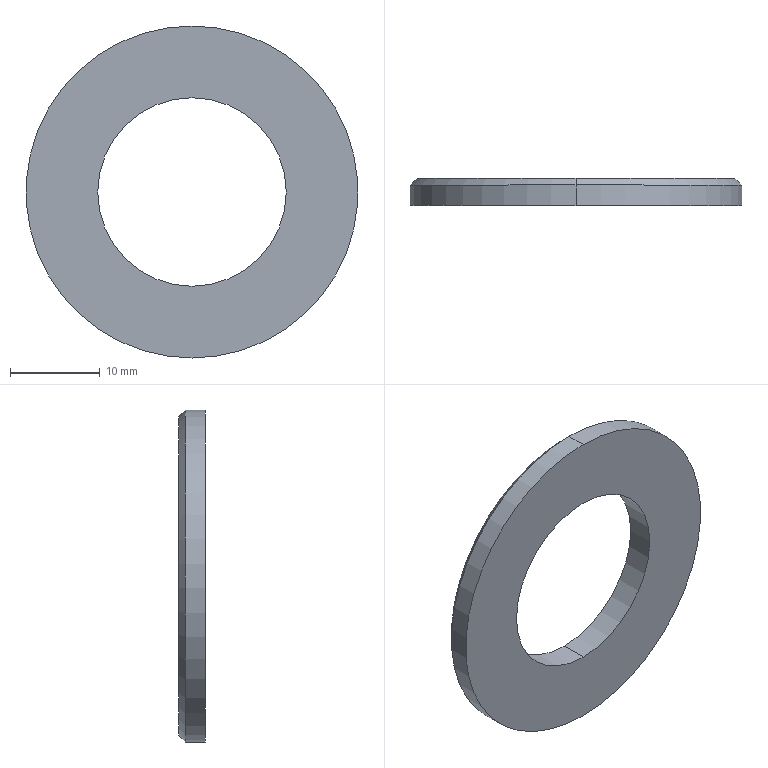Component | SolidWorks | GB_T97.2-1985FlatWasherChamferedTypeA-grade20_3-3 | 1 solid | 8 faces | box 37 x 3 x 37 mm | volume 2154 mm3 | cylinder 4 | cone 2 | plane 2 | commonest cylinder face diameters 37 x2 21 x2
build123d program:
from build123d import *


with BuildPart() as part:
    # Sketch1 → Base-Revolve (revolve)
    with BuildSketch(Plane.XY, mode=Mode.PRIVATE) as base_revolve_sk:
        Polygon((-17.75, 11.645), (-18.5, 10.895), (-18.5, 8.645), (-10.5, 8.645), (-10.5, 11.645), align=None)
    revolve(base_revolve_sk.sketch.rotate(Axis((0, 0, 0), (0, 1, 0)), 270), axis=Axis((0, 0, 0), (0, 1, 0)))


solid = part.part

# Placed as in the assembly
solid = solid.moved(Location((180, -200.645, 130), (0, 0, 0)))
STEP:
#1=CARTESIAN_POINT('',(7.087,-7.47,4.39));
#2=VERTEX_POINT('',#1);
#3=CARTESIAN_POINT('',(7.087,-7.47,5.846));
#4=VERTEX_POINT('',#3);
#5=CARTESIAN_POINT('',(7.087,-7.47,5.118));
#6=DIRECTION('',(0.,-1.,0.));
#7=DIRECTION('',(0.,0.,-1.));
#8=AXIS2_PLACEMENT_3D('',#5,#6,#7);
#9=CIRCLE('',#8,0.7283);
#10=EDGE_CURVE('',#2,#4,#9,.T.);
#11=ORIENTED_EDGE('',*,*,#10,.T.);
#12=CARTESIAN_POINT('',(7.087,-7.559,5.846));
#13=VERTEX_POINT('',#12);
#14=CARTESIAN_POINT('',(7.087,-7.899,5.846));
#15=DIRECTION('',(0.,-1.,0.));
#16=VECTOR('',#15,39.37);
#17=LINE('',#14,#16);
#18=EDGE_CURVE('',#4,#13,#17,.T.);
#19=ORIENTED_EDGE('',*,*,#18,.T.);
#20=CARTESIAN_POINT('',(7.087,-7.559,4.39));
#21=VERTEX_POINT('',#20);
#22=CARTESIAN_POINT('',(7.087,-7.559,5.118));
#23=DIRECTION('',(0.,-1.,0.));
#24=DIRECTION('',(0.,0.,-1.));
#25=AXIS2_PLACEMENT_3D('',#22,#23,#24);
#26=CIRCLE('',#25,0.7283);
#27=EDGE_CURVE('',#21,#13,#26,.T.);
#28=ORIENTED_EDGE('',*,*,#27,.F.);
#29=CARTESIAN_POINT('',(7.087,-7.899,4.39));
#30=DIRECTION('',(0.,-1.,0.));
#31=VECTOR('',#30,39.37);
#32=LINE('',#29,#31);
#33=EDGE_CURVE('',#2,#21,#32,.T.);
#34=ORIENTED_EDGE('',*,*,#33,.F.);
#35=EDGE_LOOP('',(#11,#19,#28,#34));
#36=FACE_OUTER_BOUND('',#35,.T.);
#37=CARTESIAN_POINT('',(7.087,-7.899,5.118));
#38=DIRECTION('',(0.,-1.,0.));
#39=DIRECTION('',(0.,0.,-1.));
#40=AXIS2_PLACEMENT_3D('',#37,#38,#39);
#41=CYLINDRICAL_SURFACE('',#40,0.7283);
#42=ADVANCED_FACE('',(#36),#41,.T.);
#43=CARTESIAN_POINT('',(7.087,-7.441,4.419));
#44=VERTEX_POINT('',#43);
#45=CARTESIAN_POINT('',(7.087,-7.441,5.817));
#46=VERTEX_POINT('',#45);
#47=CARTESIAN_POINT('',(7.087,-7.441,5.118));
#48=DIRECTION('',(0.,-1.,0.));
#49=DIRECTION('',(0.,0.,-1.));
#50=AXIS2_PLACEMENT_3D('',#47,#48,#49);
#51=CIRCLE('',#50,0.6988);
#52=EDGE_CURVE('',#44,#46,#51,.T.);
#53=ORIENTED_EDGE('',*,*,#52,.T.);
#54=CARTESIAN_POINT('',(7.087,-7.441,5.817));
#55=DIRECTION('',(0.,-0.7071,0.7071));
#56=VECTOR('',#55,39.37);
#57=LINE('',#54,#56);
#58=EDGE_CURVE('',#46,#4,#57,.T.);
#59=ORIENTED_EDGE('',*,*,#58,.T.);
#60=ORIENTED_EDGE('',*,*,#10,.F.);
#61=CARTESIAN_POINT('',(7.087,-7.441,4.419));
#62=DIRECTION('',(0.,-0.7071,-0.7071));
#63=VECTOR('',#62,39.37);
#64=LINE('',#61,#63);
#65=EDGE_CURVE('',#44,#2,#64,.T.);
#66=ORIENTED_EDGE('',*,*,#65,.F.);
#67=EDGE_LOOP('',(#53,#59,#60,#66));
#68=FACE_OUTER_BOUND('',#67,.T.);
#69=CARTESIAN_POINT('',(7.087,-7.441,5.118));
#70=DIRECTION('',(0.,-1.,0.));
#71=DIRECTION('',(0.,0.,-1.));
#72=AXIS2_PLACEMENT_3D('',#69,#70,#71);
#73=CONICAL_SURFACE('',#72,0.6988,0.7854);
#74=ADVANCED_FACE('',(#68),#73,.T.);
#75=CARTESIAN_POINT('',(7.087,-7.441,5.531));
#76=VERTEX_POINT('',#75);
#77=CARTESIAN_POINT('',(7.087,-7.441,4.705));
#78=VERTEX_POINT('',#77);
#79=CARTESIAN_POINT('',(7.087,-7.441,5.118));
#80=DIRECTION('',(0.,-1.,0.));
#81=DIRECTION('',(0.,0.,-1.));
#82=AXIS2_PLACEMENT_3D('',#79,#80,#81);
#83=CIRCLE('',#82,0.4134);
#84=EDGE_CURVE('',#76,#78,#83,.T.);
#85=ORIENTED_EDGE('',*,*,#84,.F.);
#86=CARTESIAN_POINT('',(7.087,-7.559,5.531));
#87=VERTEX_POINT('',#86);
#88=CARTESIAN_POINT('',(7.087,-7.899,5.531));
#89=DIRECTION('',(0.,-1.,0.));
#90=VECTOR('',#89,39.37);
#91=LINE('',#88,#90);
#92=EDGE_CURVE('',#76,#87,#91,.T.);
#93=ORIENTED_EDGE('',*,*,#92,.T.);
#94=CARTESIAN_POINT('',(7.087,-7.559,4.705));
#95=VERTEX_POINT('',#94);
#96=CARTESIAN_POINT('',(7.087,-7.559,5.118));
#97=DIRECTION('',(0.,-1.,0.));
#98=DIRECTION('',(0.,0.,-1.));
#99=AXIS2_PLACEMENT_3D('',#96,#97,#98);
#100=CIRCLE('',#99,0.4134);
#101=EDGE_CURVE('',#87,#95,#100,.T.);
#102=ORIENTED_EDGE('',*,*,#101,.T.);
#103=CARTESIAN_POINT('',(7.087,-7.899,4.705));
#104=DIRECTION('',(0.,-1.,0.));
#105=VECTOR('',#104,39.37);
#106=LINE('',#103,#105);
#107=EDGE_CURVE('',#78,#95,#106,.T.);
#108=ORIENTED_EDGE('',*,*,#107,.F.);
#109=EDGE_LOOP('',(#85,#93,#102,#108));
#110=FACE_OUTER_BOUND('',#109,.T.);
#111=CARTESIAN_POINT('',(7.087,-7.899,5.118));
#112=DIRECTION('',(0.,-1.,0.));
#113=DIRECTION('',(0.,0.,-1.));
#114=AXIS2_PLACEMENT_3D('',#111,#112,#113);
#115=CYLINDRICAL_SURFACE('',#114,0.4134);
#116=ADVANCED_FACE('',(#110),#115,.F.);
#117=ORIENTED_EDGE('',*,*,#92,.F.);
#118=CARTESIAN_POINT('',(7.087,-7.441,5.118));
#119=DIRECTION('',(0.,-1.,0.));
#120=DIRECTION('',(0.,0.,-1.));
#121=AXIS2_PLACEMENT_3D('',#118,#119,#120);
#122=CIRCLE('',#121,0.4134);
#123=EDGE_CURVE('',#78,#76,#122,.T.);
#124=ORIENTED_EDGE('',*,*,#123,.F.);
#125=ORIENTED_EDGE('',*,*,#107,.T.);
#126=CARTESIAN_POINT('',(7.087,-7.559,5.118));
#127=DIRECTION('',(0.,-1.,0.));
#128=DIRECTION('',(0.,0.,-1.));
#129=AXIS2_PLACEMENT_3D('',#126,#127,#128);
#130=CIRCLE('',#129,0.4134);
#131=EDGE_CURVE('',#95,#87,#130,.T.);
#132=ORIENTED_EDGE('',*,*,#131,.T.);
#133=EDGE_LOOP('',(#117,#124,#125,#132));
#134=FACE_OUTER_BOUND('',#133,.T.);
#135=CARTESIAN_POINT('',(7.087,-7.899,5.118));
#136=DIRECTION('',(0.,-1.,0.));
#137=DIRECTION('',(0.,0.,-1.));
#138=AXIS2_PLACEMENT_3D('',#135,#136,#137);
#139=CYLINDRICAL_SURFACE('',#138,0.4134);
#140=ADVANCED_FACE('',(#134),#139,.F.);
#141=ORIENTED_EDGE('',*,*,#52,.F.);
#142=CARTESIAN_POINT('',(7.087,-7.441,5.118));
#143=DIRECTION('',(0.,-1.,0.));
#144=DIRECTION('',(0.,0.,-1.));
#145=AXIS2_PLACEMENT_3D('',#142,#143,#144);
#146=CIRCLE('',#145,0.6988);
#147=EDGE_CURVE('',#46,#44,#146,.T.);
#148=ORIENTED_EDGE('',*,*,#147,.F.);
#149=EDGE_LOOP('',(#141,#148));
#150=FACE_OUTER_BOUND('',#149,.T.);
#151=ORIENTED_EDGE('',*,*,#123,.T.);
#152=ORIENTED_EDGE('',*,*,#84,.T.);
#153=EDGE_LOOP('',(#151,#152));
#154=FACE_BOUND('',#153,.T.);
#155=CARTESIAN_POINT('',(6.673,-7.441,5.118));
#156=DIRECTION('',(0.,-1.,0.));
#157=DIRECTION('',(0.,0.,-1.));
#158=AXIS2_PLACEMENT_3D('',#155,#156,#157);
#159=PLANE('',#158);
#160=ADVANCED_FACE('',(#150,#154),#159,.F.);
#161=ORIENTED_EDGE('',*,*,#58,.F.);
#162=ORIENTED_EDGE('',*,*,#147,.T.);
#163=ORIENTED_EDGE('',*,*,#65,.T.);
#164=CARTESIAN_POINT('',(7.087,-7.47,5.118));
#165=DIRECTION('',(0.,-1.,0.));
#166=DIRECTION('',(0.,0.,-1.));
#167=AXIS2_PLACEMENT_3D('',#164,#165,#166);
#168=CIRCLE('',#167,0.7283);
#169=EDGE_CURVE('',#4,#2,#168,.T.);
#170=ORIENTED_EDGE('',*,*,#169,.F.);
#171=EDGE_LOOP('',(#161,#162,#163,#170));
#172=FACE_OUTER_BOUND('',#171,.T.);
#173=CARTESIAN_POINT('',(7.087,-7.441,5.118));
#174=DIRECTION('',(0.,-1.,0.));
#175=DIRECTION('',(0.,0.,-1.));
#176=AXIS2_PLACEMENT_3D('',#173,#174,#175);
#177=CONICAL_SURFACE('',#176,0.6988,0.7854);
#178=ADVANCED_FACE('',(#172),#177,.T.);
#179=ORIENTED_EDGE('',*,*,#18,.F.);
#180=ORIENTED_EDGE('',*,*,#169,.T.);
#181=ORIENTED_EDGE('',*,*,#33,.T.);
#182=CARTESIAN_POINT('',(7.087,-7.559,5.118));
#183=DIRECTION('',(0.,-1.,0.));
#184=DIRECTION('',(0.,0.,-1.));
#185=AXIS2_PLACEMENT_3D('',#182,#183,#184);
#186=CIRCLE('',#185,0.7283);
#187=EDGE_CURVE('',#13,#21,#186,.T.);
#188=ORIENTED_EDGE('',*,*,#187,.F.);
#189=EDGE_LOOP('',(#179,#180,#181,#188));
#190=FACE_OUTER_BOUND('',#189,.T.);
#191=CARTESIAN_POINT('',(7.087,-7.899,5.118));
#192=DIRECTION('',(0.,-1.,0.));
#193=DIRECTION('',(0.,0.,-1.));
#194=AXIS2_PLACEMENT_3D('',#191,#192,#193);
#195=CYLINDRICAL_SURFACE('',#194,0.7283);
#196=ADVANCED_FACE('',(#190),#195,.T.);
#197=ORIENTED_EDGE('',*,*,#131,.F.);
#198=ORIENTED_EDGE('',*,*,#101,.F.);
#199=EDGE_LOOP('',(#197,#198));
#200=FACE_BOUND('',#199,.T.);
#201=ORIENTED_EDGE('',*,*,#27,.T.);
#202=ORIENTED_EDGE('',*,*,#187,.T.);
#203=EDGE_LOOP('',(#201,#202));
#204=FACE_OUTER_BOUND('',#203,.T.);
#205=CARTESIAN_POINT('',(6.673,-7.559,5.118));
#206=DIRECTION('',(0.,1.,0.));
#207=DIRECTION('',(0.,0.,1.));
#208=AXIS2_PLACEMENT_3D('',#205,#206,#207);
#209=PLANE('',#208);
#210=ADVANCED_FACE('',(#200,#204),#209,.F.);
#211=CLOSED_SHELL('',(#42,#74,#116,#140,#160,#178,#196,#210));
#212=MANIFOLD_SOLID_BREP('',#211);
#213=CARTESIAN_POINT('',(0.,0.,0.));
#214=DIRECTION('',(0.,0.,1.));
#215=DIRECTION('',(1.,0.,0.));
#216=AXIS2_PLACEMENT_3D('',#213,#214,#215);
#217=(LENGTH_UNIT()NAMED_UNIT(*)SI_UNIT($,.METRE.));
#218=LENGTH_MEASURE_WITH_UNIT(LENGTH_MEASURE(0.0254),#217);
#219=DIMENSIONAL_EXPONENTS(1.,0.,0.,0.,0.,0.,0.);
#220=(CONVERSION_BASED_UNIT('',#218)LENGTH_UNIT()NAMED_UNIT(#219));
#221=UNCERTAINTY_MEASURE_WITH_UNIT(LENGTH_MEASURE(0.00001),#220,'','');
#222=(NAMED_UNIT(*)PLANE_ANGLE_UNIT()SI_UNIT($,.RADIAN.));
#223=(NAMED_UNIT(*)SI_UNIT($,.STERADIAN.)SOLID_ANGLE_UNIT());
#224=(GEOMETRIC_REPRESENTATION_CONTEXT(3)GLOBAL_UNCERTAINTY_ASSIGNED_CONTEXT((#221))GLOBAL_UNIT_ASSIGNED_CONTEXT((#220,#222,#223))REPRESENTATION_CONTEXT('',''));
#225=ADVANCED_BREP_SHAPE_REPRESENTATION('',(#212,#216),#224);
#226=COLOUR_RGB('',0.7922,0.8196,0.9333);
#227=FILL_AREA_STYLE_COLOUR('',#226);
#228=FILL_AREA_STYLE('',(#227));
#229=SURFACE_STYLE_FILL_AREA(#228);
#230=SURFACE_SIDE_STYLE('',(#229));
#231=SURFACE_STYLE_USAGE(.BOTH.,#230);
#232=PRESENTATION_STYLE_ASSIGNMENT((#231));
#233=STYLED_ITEM('',(#232),#212);
#234=(LENGTH_UNIT()NAMED_UNIT(*)SI_UNIT($,.METRE.));
#235=LENGTH_MEASURE_WITH_UNIT(LENGTH_MEASURE(0.0254),#234);
#236=DIMENSIONAL_EXPONENTS(1.,0.,0.,0.,0.,0.,0.);
#237=(CONVERSION_BASED_UNIT('',#235)LENGTH_UNIT()NAMED_UNIT(#236));
#238=UNCERTAINTY_MEASURE_WITH_UNIT(LENGTH_MEASURE(0.00001),#237,'','');
#239=(NAMED_UNIT(*)PLANE_ANGLE_UNIT()SI_UNIT($,.RADIAN.));
#240=(NAMED_UNIT(*)SI_UNIT($,.STERADIAN.)SOLID_ANGLE_UNIT());
#241=(GEOMETRIC_REPRESENTATION_CONTEXT(3)GLOBAL_UNCERTAINTY_ASSIGNED_CONTEXT((#238))GLOBAL_UNIT_ASSIGNED_CONTEXT((#237,#239,#240))REPRESENTATION_CONTEXT('',''));
#242=MECHANICAL_DESIGN_GEOMETRIC_PRESENTATION_REPRESENTATION('',(#233),#241);
#243=PRESENTATION_LAYER_ASSIGNMENT('','',(#233));